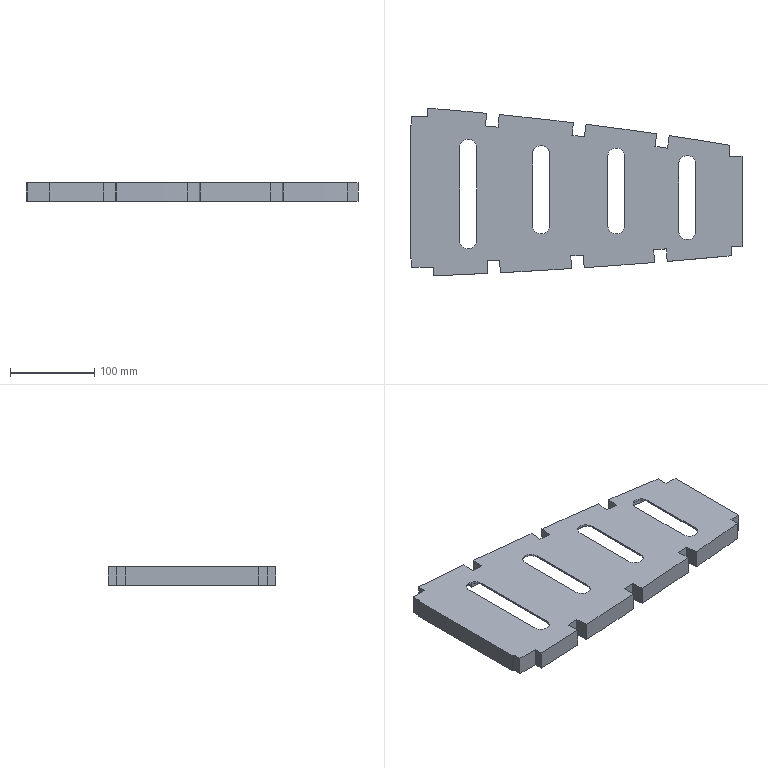Component | NX | MID_REAR_RIB | 1 solid | 99 faces | volume 164227 mm3 | plane 75 | cylinder 24 | commonest cylinder face diameters 20 x8 13198.653 x4 8411.161 x4 13194.653 x4 8407.161 x4